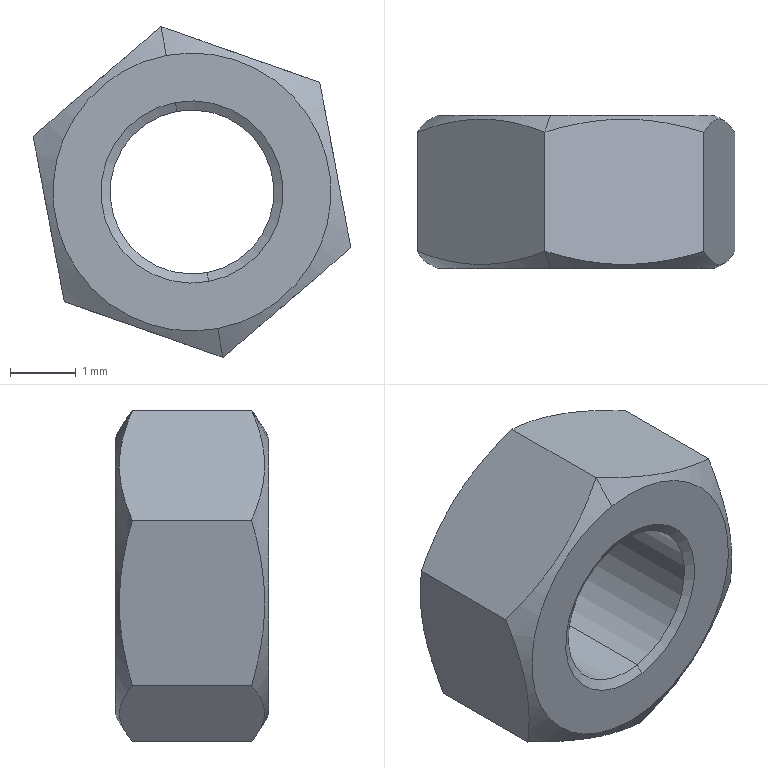Component | SolidWorks | hex nuts, style 1-grades ab gb1-10 | 1 solid | 18 faces | box 4.84 x 2.33 x 5.04 mm | volume 28 mm3 | cone 8 | plane 8 | cylinder 2 | commonest cylinder face diameters 2.5 x2
STEP:
#1=COLOUR_RGB('',0.7922,0.8196,0.9333);
#2=FILL_AREA_STYLE_COLOUR('',#1);
#3=FILL_AREA_STYLE('',(#2));
#4=SURFACE_STYLE_FILL_AREA(#3);
#5=SURFACE_SIDE_STYLE('',(#4));
#6=SURFACE_STYLE_USAGE(.BOTH.,#5);
#7=PRESENTATION_STYLE_ASSIGNMENT((#6));
#8=CARTESIAN_POINT('',(1.085,-0.2477,2.73));
#9=VERTEX_POINT('',#8);
#10=CARTESIAN_POINT('',(1.067,-0.2477,2.827));
#11=VERTEX_POINT('',#10);
#12=CARTESIAN_POINT('',(1.076,-0.2477,2.779));
#13=DIRECTION('',(-0.,-1.,-0.));
#14=DIRECTION('',(-0.1846,0.,0.9828));
#15=AXIS2_PLACEMENT_3D('',#12,#13,#14);
#16=CIRCLE('',#15,0.04921);
#17=EDGE_CURVE('',#9,#11,#16,.T.);
#18=ORIENTED_EDGE('',*,*,#17,.F.);
#19=CARTESIAN_POINT('',(1.086,-0.2509,2.725));
#20=VERTEX_POINT('',#19);
#21=CARTESIAN_POINT('',(1.085,-0.2477,2.73));
#22=DIRECTION('',(0.1598,-0.5,-0.8511));
#23=VECTOR('',#22,39.37);
#24=LINE('',#21,#23);
#25=EDGE_CURVE('',#9,#20,#24,.T.);
#26=ORIENTED_EDGE('',*,*,#25,.T.);
#27=CARTESIAN_POINT('',(1.066,-0.2509,2.833));
#28=VERTEX_POINT('',#27);
#29=CARTESIAN_POINT('',(1.076,-0.2509,2.779));
#30=DIRECTION('',(0.,1.,0.));
#31=DIRECTION('',(-0.1846,0.,0.9828));
#32=AXIS2_PLACEMENT_3D('',#29,#30,#31);
#33=CIRCLE('',#32,0.05468);
#34=EDGE_CURVE('',#28,#20,#33,.T.);
#35=ORIENTED_EDGE('',*,*,#34,.F.);
#36=CARTESIAN_POINT('',(1.067,-0.2477,2.827));
#37=DIRECTION('',(-0.1598,-0.5,0.8511));
#38=VECTOR('',#37,39.37);
#39=LINE('',#36,#38);
#40=EDGE_CURVE('',#11,#28,#39,.T.);
#41=ORIENTED_EDGE('',*,*,#40,.F.);
#42=EDGE_LOOP('',(#18,#26,#35,#41));
#43=FACE_OUTER_BOUND('',#42,.T.);
#44=CARTESIAN_POINT('',(1.076,-0.2477,2.779));
#45=DIRECTION('',(-0.,-1.,-0.));
#46=DIRECTION('',(-0.1846,0.,0.9828));
#47=AXIS2_PLACEMENT_3D('',#44,#45,#46);
#48=CONICAL_SURFACE('',#47,0.04921,1.047);
#49=ADVANCED_FACE('',(#43),#48,.F.);
#50=CARTESIAN_POINT('',(1.067,-0.1645,2.827));
#51=VERTEX_POINT('',#50);
#52=CARTESIAN_POINT('',(1.085,-0.1645,2.73));
#53=VERTEX_POINT('',#52);
#54=CARTESIAN_POINT('',(1.076,-0.1645,2.779));
#55=DIRECTION('',(0.,1.,0.));
#56=DIRECTION('',(-0.1846,0.,0.9828));
#57=AXIS2_PLACEMENT_3D('',#54,#55,#56);
#58=CIRCLE('',#57,0.04921);
#59=EDGE_CURVE('',#51,#53,#58,.T.);
#60=ORIENTED_EDGE('',*,*,#59,.F.);
#61=CARTESIAN_POINT('',(1.066,-0.159,2.83));
#62=VERTEX_POINT('',#61);
#63=CARTESIAN_POINT('',(1.066,-0.159,2.83));
#64=DIRECTION('',(-0.09228,0.866,0.4914));
#65=VECTOR('',#64,39.37);
#66=LINE('',#63,#65);
#67=EDGE_CURVE('',#51,#62,#66,.T.);
#68=ORIENTED_EDGE('',*,*,#67,.T.);
#69=CARTESIAN_POINT('',(1.085,-0.159,2.727));
#70=VERTEX_POINT('',#69);
#71=CARTESIAN_POINT('',(1.076,-0.159,2.779));
#72=DIRECTION('',(-0.,-1.,-0.));
#73=DIRECTION('',(-0.1846,0.,0.9828));
#74=AXIS2_PLACEMENT_3D('',#71,#72,#73);
#75=CIRCLE('',#74,0.05237);
#76=EDGE_CURVE('',#70,#62,#75,.T.);
#77=ORIENTED_EDGE('',*,*,#76,.F.);
#78=CARTESIAN_POINT('',(1.085,-0.159,2.727));
#79=DIRECTION('',(0.09228,0.866,-0.4914));
#80=VECTOR('',#79,39.37);
#81=LINE('',#78,#80);
#82=EDGE_CURVE('',#53,#70,#81,.T.);
#83=ORIENTED_EDGE('',*,*,#82,.F.);
#84=EDGE_LOOP('',(#60,#68,#77,#83));
#85=FACE_OUTER_BOUND('',#84,.T.);
#86=CARTESIAN_POINT('',(1.076,-0.159,2.779));
#87=DIRECTION('',(0.,1.,0.));
#88=DIRECTION('',(0.1846,0.,-0.9828));
#89=AXIS2_PLACEMENT_3D('',#86,#87,#88);
#90=CONICAL_SURFACE('',#89,0.05237,0.5236);
#91=ADVANCED_FACE('',(#85),#90,.F.);
#92=CARTESIAN_POINT('',(1.091,-0.2509,2.697));
#93=VERTEX_POINT('',#92);
#94=CARTESIAN_POINT('',(1.06,-0.2509,2.861));
#95=VERTEX_POINT('',#94);
#96=CARTESIAN_POINT('',(1.076,-0.2509,2.779));
#97=DIRECTION('',(0.,1.,0.));
#98=DIRECTION('',(0.1846,0.,-0.9828));
#99=AXIS2_PLACEMENT_3D('',#96,#97,#98);
#100=CIRCLE('',#99,0.08339);
#101=EDGE_CURVE('',#93,#95,#100,.T.);
#102=ORIENTED_EDGE('',*,*,#101,.T.);
#103=CARTESIAN_POINT('',(1.057,-0.2407,2.878));
#104=VERTEX_POINT('',#103);
#105=CARTESIAN_POINT('',(1.06,-0.2509,2.861));
#106=DIRECTION('',(-0.1598,0.5,0.8511));
#107=VECTOR('',#106,39.37);
#108=LINE('',#105,#107);
#109=EDGE_CURVE('',#95,#104,#108,.T.);
#110=ORIENTED_EDGE('',*,*,#109,.T.);
#111=CARTESIAN_POINT('',(0.9805,-0.2407,2.812));
#112=VERTEX_POINT('',#111);
#113=CARTESIAN_POINT('',(1.057,-0.2407,2.878));
#114=CARTESIAN_POINT('',(1.045,-0.2455,2.867));
#115=CARTESIAN_POINT('',(1.032,-0.2485,2.856));
#116=CARTESIAN_POINT('',(1.012,-0.2485,2.84));
#117=CARTESIAN_POINT('',(1.006,-0.2478,2.834));
#118=CARTESIAN_POINT('',(0.9931,-0.245,2.823));
#119=CARTESIAN_POINT('',(0.9868,-0.2431,2.818));
#120=CARTESIAN_POINT('',(0.9805,-0.2407,2.812));
#121=B_SPLINE_CURVE_WITH_KNOTS('',3,(#113,#114,#115,#116,#117,#118,#119,#120),.UNSPECIFIED.,.F.,.F.,(4,2,2,4),(0.00000007,0.001296,0.001944,0.002592),.UNSPECIFIED.);
#122=EDGE_CURVE('',#104,#112,#121,.T.);
#123=ORIENTED_EDGE('',*,*,#122,.T.);
#124=CARTESIAN_POINT('',(0.9992,-0.2407,2.713));
#125=VERTEX_POINT('',#124);
#126=CARTESIAN_POINT('',(0.9805,-0.2407,2.812));
#127=CARTESIAN_POINT('',(0.982,-0.2431,2.804));
#128=CARTESIAN_POINT('',(0.9836,-0.245,2.796));
#129=CARTESIAN_POINT('',(0.9867,-0.2478,2.78));
#130=CARTESIAN_POINT('',(0.9883,-0.2485,2.771));
#131=CARTESIAN_POINT('',(0.9914,-0.2485,2.754));
#132=CARTESIAN_POINT('',(0.993,-0.2478,2.746));
#133=CARTESIAN_POINT('',(0.9961,-0.2451,2.729));
#134=CARTESIAN_POINT('',(0.9977,-0.2431,2.721));
#135=CARTESIAN_POINT('',(0.9992,-0.2407,2.713));
#136=B_SPLINE_CURVE_WITH_KNOTS('',3,(#126,#127,#128,#129,#130,#131,#132,#133,#134,#135),.UNSPECIFIED.,.F.,.F.,(4,2,2,2,4),(0.0009504,0.001598,0.002245,0.002893,0.00354),.UNSPECIFIED.);
#137=EDGE_CURVE('',#112,#125,#136,.T.);
#138=ORIENTED_EDGE('',*,*,#137,.T.);
#139=CARTESIAN_POINT('',(1.094,-0.2407,2.679));
#140=VERTEX_POINT('',#139);
#141=CARTESIAN_POINT('',(0.9992,-0.2407,2.713));
#142=CARTESIAN_POINT('',(1.015,-0.2455,2.708));
#143=CARTESIAN_POINT('',(1.031,-0.2485,2.702));
#144=CARTESIAN_POINT('',(1.055,-0.2485,2.693));
#145=CARTESIAN_POINT('',(1.063,-0.2478,2.691));
#146=CARTESIAN_POINT('',(1.079,-0.245,2.685));
#147=CARTESIAN_POINT('',(1.087,-0.2431,2.682));
#148=CARTESIAN_POINT('',(1.094,-0.2407,2.679));
#149=B_SPLINE_CURVE_WITH_KNOTS('',3,(#141,#142,#143,#144,#145,#146,#147,#148),.UNSPECIFIED.,.F.,.F.,(4,2,2,4),(0.00000007,0.001296,0.001944,0.002592),.UNSPECIFIED.);
#150=EDGE_CURVE('',#125,#140,#149,.T.);
#151=ORIENTED_EDGE('',*,*,#150,.T.);
#152=CARTESIAN_POINT('',(1.091,-0.2509,2.697));
#153=DIRECTION('',(0.1598,0.5,-0.8511));
#154=VECTOR('',#153,39.37);
#155=LINE('',#152,#154);
#156=EDGE_CURVE('',#93,#140,#155,.T.);
#157=ORIENTED_EDGE('',*,*,#156,.F.);
#158=EDGE_LOOP('',(#102,#110,#123,#138,#151,#157));
#159=FACE_OUTER_BOUND('',#158,.T.);
#160=CARTESIAN_POINT('',(1.076,-0.2509,2.779));
#161=DIRECTION('',(0.,1.,0.));
#162=DIRECTION('',(0.1846,0.,-0.9828));
#163=AXIS2_PLACEMENT_3D('',#160,#161,#162);
#164=CONICAL_SURFACE('',#163,0.08339,1.047);
#165=ADVANCED_FACE('',(#159),#164,.T.);
#166=CARTESIAN_POINT('',(1.091,-0.159,2.697));
#167=VERTEX_POINT('',#166);
#168=CARTESIAN_POINT('',(1.06,-0.159,2.861));
#169=VERTEX_POINT('',#168);
#170=CARTESIAN_POINT('',(1.076,-0.159,2.779));
#171=DIRECTION('',(0.,1.,0.));
#172=DIRECTION('',(0.1846,0.,-0.9828));
#173=AXIS2_PLACEMENT_3D('',#170,#171,#172);
#174=CIRCLE('',#173,0.08339);
#175=EDGE_CURVE('',#167,#169,#174,.T.);
#176=ORIENTED_EDGE('',*,*,#175,.F.);
#177=CARTESIAN_POINT('',(1.094,-0.1692,2.679));
#178=VERTEX_POINT('',#177);
#179=CARTESIAN_POINT('',(1.094,-0.1692,2.679));
#180=DIRECTION('',(0.1598,-0.5,-0.8511));
#181=VECTOR('',#180,39.37);
#182=LINE('',#179,#181);
#183=EDGE_CURVE('',#167,#178,#182,.T.);
#184=ORIENTED_EDGE('',*,*,#183,.T.);
#185=CARTESIAN_POINT('',(0.9992,-0.1692,2.713));
#186=VERTEX_POINT('',#185);
#187=CARTESIAN_POINT('',(1.094,-0.1692,2.679));
#188=CARTESIAN_POINT('',(1.079,-0.1644,2.685));
#189=CARTESIAN_POINT('',(1.063,-0.1614,2.691));
#190=CARTESIAN_POINT('',(1.039,-0.1614,2.699));
#191=CARTESIAN_POINT('',(1.031,-0.1621,2.702));
#192=CARTESIAN_POINT('',(1.015,-0.1648,2.707));
#193=CARTESIAN_POINT('',(1.007,-0.1668,2.71));
#194=CARTESIAN_POINT('',(0.9992,-0.1692,2.713));
#195=B_SPLINE_CURVE_WITH_KNOTS('',3,(#187,#188,#189,#190,#191,#192,#193,#194),.UNSPECIFIED.,.F.,.F.,(4,2,2,4),(0.00000007,0.001296,0.001944,0.002592),.UNSPECIFIED.);
#196=EDGE_CURVE('',#178,#186,#195,.T.);
#197=ORIENTED_EDGE('',*,*,#196,.T.);
#198=CARTESIAN_POINT('',(0.9805,-0.1692,2.812));
#199=VERTEX_POINT('',#198);
#200=CARTESIAN_POINT('',(0.9992,-0.1692,2.713));
#201=CARTESIAN_POINT('',(0.9977,-0.1668,2.721));
#202=CARTESIAN_POINT('',(0.9961,-0.1648,2.729));
#203=CARTESIAN_POINT('',(0.993,-0.1621,2.746));
#204=CARTESIAN_POINT('',(0.9914,-0.1614,2.754));
#205=CARTESIAN_POINT('',(0.9883,-0.1614,2.771));
#206=CARTESIAN_POINT('',(0.9867,-0.1621,2.78));
#207=CARTESIAN_POINT('',(0.9836,-0.1649,2.796));
#208=CARTESIAN_POINT('',(0.982,-0.1668,2.804));
#209=CARTESIAN_POINT('',(0.9805,-0.1692,2.812));
#210=B_SPLINE_CURVE_WITH_KNOTS('',3,(#200,#201,#202,#203,#204,#205,#206,#207,#208,#209),.UNSPECIFIED.,.F.,.F.,(4,2,2,2,4),(0.00228,0.002929,0.003578,0.004227,0.004876),.UNSPECIFIED.);
#211=EDGE_CURVE('',#186,#199,#210,.T.);
#212=ORIENTED_EDGE('',*,*,#211,.T.);
#213=CARTESIAN_POINT('',(1.057,-0.1692,2.878));
#214=VERTEX_POINT('',#213);
#215=CARTESIAN_POINT('',(0.9805,-0.1692,2.812));
#216=CARTESIAN_POINT('',(0.993,-0.1644,2.823));
#217=CARTESIAN_POINT('',(1.006,-0.1614,2.834));
#218=CARTESIAN_POINT('',(1.025,-0.1614,2.851));
#219=CARTESIAN_POINT('',(1.032,-0.1621,2.856));
#220=CARTESIAN_POINT('',(1.045,-0.1648,2.867));
#221=CARTESIAN_POINT('',(1.051,-0.1668,2.873));
#222=CARTESIAN_POINT('',(1.057,-0.1692,2.878));
#223=B_SPLINE_CURVE_WITH_KNOTS('',3,(#215,#216,#217,#218,#219,#220,#221,#222),.UNSPECIFIED.,.F.,.F.,(4,2,2,4),(0.00000007,0.001296,0.001944,0.002592),.UNSPECIFIED.);
#224=EDGE_CURVE('',#199,#214,#223,.T.);
#225=ORIENTED_EDGE('',*,*,#224,.T.);
#226=CARTESIAN_POINT('',(1.057,-0.1692,2.878));
#227=DIRECTION('',(-0.1598,-0.5,0.8511));
#228=VECTOR('',#227,39.37);
#229=LINE('',#226,#228);
#230=EDGE_CURVE('',#169,#214,#229,.T.);
#231=ORIENTED_EDGE('',*,*,#230,.F.);
#232=EDGE_LOOP('',(#176,#184,#197,#212,#225,#231));
#233=FACE_OUTER_BOUND('',#232,.T.);
#234=CARTESIAN_POINT('',(1.076,-0.1692,2.779));
#235=DIRECTION('',(-0.,-1.,-0.));
#236=DIRECTION('',(-0.1846,0.,0.9828));
#237=AXIS2_PLACEMENT_3D('',#234,#235,#236);
#238=CONICAL_SURFACE('',#237,0.101,1.047);
#239=ADVANCED_FACE('',(#233),#238,.T.);
#240=ORIENTED_EDGE('',*,*,#59,.T.);
#241=CARTESIAN_POINT('',(1.085,-0.159,2.73));
#242=DIRECTION('',(-0.,-1.,-0.));
#243=VECTOR('',#242,39.37);
#244=LINE('',#241,#243);
#245=EDGE_CURVE('',#53,#9,#244,.T.);
#246=ORIENTED_EDGE('',*,*,#245,.T.);
#247=ORIENTED_EDGE('',*,*,#17,.T.);
#248=CARTESIAN_POINT('',(1.067,-0.159,2.827));
#249=DIRECTION('',(-0.,-1.,-0.));
#250=VECTOR('',#249,39.37);
#251=LINE('',#248,#250);
#252=EDGE_CURVE('',#51,#11,#251,.T.);
#253=ORIENTED_EDGE('',*,*,#252,.F.);
#254=EDGE_LOOP('',(#240,#246,#247,#253));
#255=FACE_OUTER_BOUND('',#254,.T.);
#256=CARTESIAN_POINT('',(1.076,-0.159,2.779));
#257=DIRECTION('',(-0.,-1.,-0.));
#258=DIRECTION('',(-0.1846,0.,0.9828));
#259=AXIS2_PLACEMENT_3D('',#256,#257,#258);
#260=CYLINDRICAL_SURFACE('',#259,0.04921);
#261=ADVANCED_FACE('',(#255),#260,.F.);
#262=CARTESIAN_POINT('',(1.152,-0.2407,2.845));
#263=VERTEX_POINT('',#262);
#264=CARTESIAN_POINT('',(1.152,-0.2407,2.845));
#265=CARTESIAN_POINT('',(1.137,-0.2455,2.85));
#266=CARTESIAN_POINT('',(1.121,-0.2485,2.856));
#267=CARTESIAN_POINT('',(1.097,-0.2485,2.864));
#268=CARTESIAN_POINT('',(1.089,-0.2478,2.867));
#269=CARTESIAN_POINT('',(1.073,-0.245,2.873));
#270=CARTESIAN_POINT('',(1.065,-0.2431,2.875));
#271=CARTESIAN_POINT('',(1.057,-0.2407,2.878));
#272=B_SPLINE_CURVE_WITH_KNOTS('',3,(#264,#265,#266,#267,#268,#269,#270,#271),.UNSPECIFIED.,.F.,.F.,(4,2,2,4),(0.00000007,0.001296,0.001944,0.002592),.UNSPECIFIED.);
#273=EDGE_CURVE('',#263,#104,#272,.T.);
#274=ORIENTED_EDGE('',*,*,#273,.F.);
#275=CARTESIAN_POINT('',(1.152,-0.1692,2.845));
#276=VERTEX_POINT('',#275);
#277=CARTESIAN_POINT('',(1.152,-0.159,2.845));
#278=DIRECTION('',(-0.,-1.,-0.));
#279=VECTOR('',#278,39.37);
#280=LINE('',#277,#279);
#281=EDGE_CURVE('',#276,#263,#280,.T.);
#282=ORIENTED_EDGE('',*,*,#281,.F.);
#283=CARTESIAN_POINT('',(1.057,-0.1692,2.878));
#284=CARTESIAN_POINT('',(1.073,-0.1644,2.873));
#285=CARTESIAN_POINT('',(1.089,-0.1614,2.867));
#286=CARTESIAN_POINT('',(1.113,-0.1614,2.859));
#287=CARTESIAN_POINT('',(1.121,-0.1621,2.856));
#288=CARTESIAN_POINT('',(1.137,-0.1648,2.85));
#289=CARTESIAN_POINT('',(1.145,-0.1668,2.847));
#290=CARTESIAN_POINT('',(1.152,-0.1692,2.845));
#291=B_SPLINE_CURVE_WITH_KNOTS('',3,(#283,#284,#285,#286,#287,#288,#289,#290),.UNSPECIFIED.,.F.,.F.,(4,2,2,4),(0.00000007,0.001296,0.001944,0.002592),.UNSPECIFIED.);
#292=EDGE_CURVE('',#214,#276,#291,.T.);
#293=ORIENTED_EDGE('',*,*,#292,.F.);
#294=CARTESIAN_POINT('',(1.057,-0.159,2.878));
#295=DIRECTION('',(-0.,-1.,-0.));
#296=VECTOR('',#295,39.37);
#297=LINE('',#294,#296);
#298=EDGE_CURVE('',#214,#104,#297,.T.);
#299=ORIENTED_EDGE('',*,*,#298,.T.);
#300=EDGE_LOOP('',(#274,#282,#293,#299));
#301=FACE_OUTER_BOUND('',#300,.T.);
#302=CARTESIAN_POINT('',(1.152,-0.159,2.845));
#303=DIRECTION('',(0.3316,0.,0.9434));
#304=DIRECTION('',(-0.9434,0.,0.3316));
#305=AXIS2_PLACEMENT_3D('',#302,#303,#304);
#306=PLANE('',#305);
#307=ADVANCED_FACE('',(#301),#306,.T.);
#308=CARTESIAN_POINT('',(1.171,-0.2407,2.745));
#309=VERTEX_POINT('',#308);
#310=CARTESIAN_POINT('',(1.171,-0.2407,2.745));
#311=CARTESIAN_POINT('',(1.17,-0.2431,2.753));
#312=CARTESIAN_POINT('',(1.168,-0.2451,2.762));
#313=CARTESIAN_POINT('',(1.165,-0.2478,2.778));
#314=CARTESIAN_POINT('',(1.163,-0.2485,2.787));
#315=CARTESIAN_POINT('',(1.16,-0.2485,2.803));
#316=CARTESIAN_POINT('',(1.159,-0.2478,2.812));
#317=CARTESIAN_POINT('',(1.156,-0.245,2.828));
#318=CARTESIAN_POINT('',(1.154,-0.2431,2.837));
#319=CARTESIAN_POINT('',(1.152,-0.2407,2.845));
#320=B_SPLINE_CURVE_WITH_KNOTS('',3,(#310,#311,#312,#313,#314,#315,#316,#317,#318,#319),.UNSPECIFIED.,.F.,.F.,(4,2,2,2,4),(0.00228,0.002929,0.003578,0.004227,0.004876),.UNSPECIFIED.);
#321=EDGE_CURVE('',#309,#263,#320,.T.);
#322=ORIENTED_EDGE('',*,*,#321,.F.);
#323=CARTESIAN_POINT('',(1.171,-0.1692,2.745));
#324=VERTEX_POINT('',#323);
#325=CARTESIAN_POINT('',(1.171,-0.159,2.745));
#326=DIRECTION('',(-0.,-1.,-0.));
#327=VECTOR('',#326,39.37);
#328=LINE('',#325,#327);
#329=EDGE_CURVE('',#324,#309,#328,.T.);
#330=ORIENTED_EDGE('',*,*,#329,.F.);
#331=CARTESIAN_POINT('',(1.152,-0.1692,2.845));
#332=CARTESIAN_POINT('',(1.154,-0.1668,2.837));
#333=CARTESIAN_POINT('',(1.156,-0.1649,2.828));
#334=CARTESIAN_POINT('',(1.159,-0.1621,2.812));
#335=CARTESIAN_POINT('',(1.16,-0.1614,2.803));
#336=CARTESIAN_POINT('',(1.163,-0.1614,2.787));
#337=CARTESIAN_POINT('',(1.165,-0.1621,2.778));
#338=CARTESIAN_POINT('',(1.168,-0.1648,2.762));
#339=CARTESIAN_POINT('',(1.17,-0.1668,2.753));
#340=CARTESIAN_POINT('',(1.171,-0.1692,2.745));
#341=B_SPLINE_CURVE_WITH_KNOTS('',3,(#331,#332,#333,#334,#335,#336,#337,#338,#339,#340),.UNSPECIFIED.,.F.,.F.,(4,2,2,2,4),(0.0009504,0.001598,0.002245,0.002893,0.00354),.UNSPECIFIED.);
#342=EDGE_CURVE('',#276,#324,#341,.T.);
#343=ORIENTED_EDGE('',*,*,#342,.F.);
#344=ORIENTED_EDGE('',*,*,#281,.T.);
#345=EDGE_LOOP('',(#322,#330,#343,#344));
#346=FACE_OUTER_BOUND('',#345,.T.);
#347=CARTESIAN_POINT('',(1.171,-0.159,2.745));
#348=DIRECTION('',(0.9828,-0.,0.1846));
#349=DIRECTION('',(0.,1.,0.));
#350=AXIS2_PLACEMENT_3D('',#347,#348,#349);
#351=PLANE('',#350);
#352=ADVANCED_FACE('',(#346),#351,.T.);
#353=CARTESIAN_POINT('',(1.094,-0.2407,2.679));
#354=CARTESIAN_POINT('',(1.107,-0.2455,2.69));
#355=CARTESIAN_POINT('',(1.12,-0.2485,2.701));
#356=CARTESIAN_POINT('',(1.139,-0.2485,2.718));
#357=CARTESIAN_POINT('',(1.146,-0.2478,2.724));
#358=CARTESIAN_POINT('',(1.159,-0.245,2.734));
#359=CARTESIAN_POINT('',(1.165,-0.2431,2.74));
#360=CARTESIAN_POINT('',(1.171,-0.2407,2.745));
#361=B_SPLINE_CURVE_WITH_KNOTS('',3,(#353,#354,#355,#356,#357,#358,#359,#360),.UNSPECIFIED.,.F.,.F.,(4,2,2,4),(0.00000007,0.001296,0.001944,0.002592),.UNSPECIFIED.);
#362=EDGE_CURVE('',#140,#309,#361,.T.);
#363=ORIENTED_EDGE('',*,*,#362,.F.);
#364=CARTESIAN_POINT('',(1.094,-0.159,2.679));
#365=DIRECTION('',(-0.,-1.,-0.));
#366=VECTOR('',#365,39.37);
#367=LINE('',#364,#366);
#368=EDGE_CURVE('',#178,#140,#367,.T.);
#369=ORIENTED_EDGE('',*,*,#368,.F.);
#370=CARTESIAN_POINT('',(1.171,-0.1692,2.745));
#371=CARTESIAN_POINT('',(1.159,-0.1644,2.735));
#372=CARTESIAN_POINT('',(1.146,-0.1614,2.724));
#373=CARTESIAN_POINT('',(1.126,-0.1614,2.707));
#374=CARTESIAN_POINT('',(1.12,-0.1621,2.701));
#375=CARTESIAN_POINT('',(1.107,-0.1648,2.69));
#376=CARTESIAN_POINT('',(1.101,-0.1668,2.685));
#377=CARTESIAN_POINT('',(1.094,-0.1692,2.679));
#378=B_SPLINE_CURVE_WITH_KNOTS('',3,(#370,#371,#372,#373,#374,#375,#376,#377),.UNSPECIFIED.,.F.,.F.,(4,2,2,4),(0.00000007,0.001296,0.001944,0.002592),.UNSPECIFIED.);
#379=EDGE_CURVE('',#324,#178,#378,.T.);
#380=ORIENTED_EDGE('',*,*,#379,.F.);
#381=ORIENTED_EDGE('',*,*,#329,.T.);
#382=EDGE_LOOP('',(#363,#369,#380,#381));
#383=FACE_OUTER_BOUND('',#382,.T.);
#384=CARTESIAN_POINT('',(1.094,-0.159,2.679));
#385=DIRECTION('',(0.6512,-0.,-0.7589));
#386=DIRECTION('',(0.7589,-0.,0.6512));
#387=AXIS2_PLACEMENT_3D('',#384,#385,#386);
#388=PLANE('',#387);
#389=ADVANCED_FACE('',(#383),#388,.T.);
#390=ORIENTED_EDGE('',*,*,#150,.F.);
#391=CARTESIAN_POINT('',(0.9992,-0.159,2.713));
#392=DIRECTION('',(-0.,-1.,-0.));
#393=VECTOR('',#392,39.37);
#394=LINE('',#391,#393);
#395=EDGE_CURVE('',#186,#125,#394,.T.);
#396=ORIENTED_EDGE('',*,*,#395,.F.);
#397=ORIENTED_EDGE('',*,*,#196,.F.);
#398=ORIENTED_EDGE('',*,*,#368,.T.);
#399=EDGE_LOOP('',(#390,#396,#397,#398));
#400=FACE_OUTER_BOUND('',#399,.T.);
#401=CARTESIAN_POINT('',(0.9992,-0.159,2.713));
#402=DIRECTION('',(-0.3316,-0.,-0.9434));
#403=DIRECTION('',(0.9434,-0.,-0.3316));
#404=AXIS2_PLACEMENT_3D('',#401,#402,#403);
#405=PLANE('',#404);
#406=ADVANCED_FACE('',(#400),#405,.T.);
#407=ORIENTED_EDGE('',*,*,#137,.F.);
#408=CARTESIAN_POINT('',(0.9805,-0.159,2.812));
#409=DIRECTION('',(-0.,-1.,-0.));
#410=VECTOR('',#409,39.37);
#411=LINE('',#408,#410);
#412=EDGE_CURVE('',#199,#112,#411,.T.);
#413=ORIENTED_EDGE('',*,*,#412,.F.);
#414=ORIENTED_EDGE('',*,*,#211,.F.);
#415=ORIENTED_EDGE('',*,*,#395,.T.);
#416=EDGE_LOOP('',(#407,#413,#414,#415));
#417=FACE_OUTER_BOUND('',#416,.T.);
#418=CARTESIAN_POINT('',(0.9805,-0.159,2.812));
#419=DIRECTION('',(-0.9828,0.,-0.1846));
#420=DIRECTION('',(-0.,-1.,-0.));
#421=AXIS2_PLACEMENT_3D('',#418,#419,#420);
#422=PLANE('',#421);
#423=ADVANCED_FACE('',(#417),#422,.T.);
#424=ORIENTED_EDGE('',*,*,#122,.F.);
#425=ORIENTED_EDGE('',*,*,#298,.F.);
#426=ORIENTED_EDGE('',*,*,#224,.F.);
#427=ORIENTED_EDGE('',*,*,#412,.T.);
#428=EDGE_LOOP('',(#424,#425,#426,#427));
#429=FACE_OUTER_BOUND('',#428,.T.);
#430=CARTESIAN_POINT('',(1.057,-0.159,2.878));
#431=DIRECTION('',(-0.6512,0.,0.7589));
#432=DIRECTION('',(-0.7589,0.,-0.6512));
#433=AXIS2_PLACEMENT_3D('',#430,#431,#432);
#434=PLANE('',#433);
#435=ADVANCED_FACE('',(#429),#434,.T.);
#436=ORIENTED_EDGE('',*,*,#76,.T.);
#437=CARTESIAN_POINT('',(1.076,-0.159,2.779));
#438=DIRECTION('',(-0.,-1.,-0.));
#439=DIRECTION('',(-0.1846,0.,0.9828));
#440=AXIS2_PLACEMENT_3D('',#437,#438,#439);
#441=CIRCLE('',#440,0.05237);
#442=EDGE_CURVE('',#62,#70,#441,.T.);
#443=ORIENTED_EDGE('',*,*,#442,.T.);
#444=EDGE_LOOP('',(#436,#443));
#445=FACE_BOUND('',#444,.T.);
#446=CARTESIAN_POINT('',(1.076,-0.159,2.779));
#447=DIRECTION('',(0.,1.,0.));
#448=DIRECTION('',(0.1846,0.,-0.9828));
#449=AXIS2_PLACEMENT_3D('',#446,#447,#448);
#450=CIRCLE('',#449,0.08339);
#451=EDGE_CURVE('',#169,#167,#450,.T.);
#452=ORIENTED_EDGE('',*,*,#451,.T.);
#453=ORIENTED_EDGE('',*,*,#175,.T.);
#454=EDGE_LOOP('',(#452,#453));
#455=FACE_OUTER_BOUND('',#454,.T.);
#456=CARTESIAN_POINT('',(1.057,-0.159,2.878));
#457=DIRECTION('',(-0.,-1.,0.));
#458=DIRECTION('',(-0.1846,0.,0.9828));
#459=AXIS2_PLACEMENT_3D('',#456,#457,#458);
#460=PLANE('',#459);
#461=ADVANCED_FACE('',(#445,#455),#460,.F.);
#462=ORIENTED_EDGE('',*,*,#34,.T.);
#463=CARTESIAN_POINT('',(1.076,-0.2509,2.779));
#464=DIRECTION('',(0.,1.,0.));
#465=DIRECTION('',(-0.1846,0.,0.9828));
#466=AXIS2_PLACEMENT_3D('',#463,#464,#465);
#467=CIRCLE('',#466,0.05468);
#468=EDGE_CURVE('',#20,#28,#467,.T.);
#469=ORIENTED_EDGE('',*,*,#468,.T.);
#470=EDGE_LOOP('',(#462,#469));
#471=FACE_BOUND('',#470,.T.);
#472=ORIENTED_EDGE('',*,*,#101,.F.);
#473=CARTESIAN_POINT('',(1.076,-0.2509,2.779));
#474=DIRECTION('',(0.,1.,0.));
#475=DIRECTION('',(0.1846,0.,-0.9828));
#476=AXIS2_PLACEMENT_3D('',#473,#474,#475);
#477=CIRCLE('',#476,0.08339);
#478=EDGE_CURVE('',#95,#93,#477,.T.);
#479=ORIENTED_EDGE('',*,*,#478,.F.);
#480=EDGE_LOOP('',(#472,#479));
#481=FACE_OUTER_BOUND('',#480,.T.);
#482=CARTESIAN_POINT('',(1.057,-0.2509,2.878));
#483=DIRECTION('',(-0.,-1.,0.));
#484=DIRECTION('',(-0.1846,0.,0.9828));
#485=AXIS2_PLACEMENT_3D('',#482,#483,#484);
#486=PLANE('',#485);
#487=ADVANCED_FACE('',(#471,#481),#486,.T.);
#488=ORIENTED_EDGE('',*,*,#245,.F.);
#489=CARTESIAN_POINT('',(1.076,-0.1645,2.779));
#490=DIRECTION('',(0.,1.,0.));
#491=DIRECTION('',(-0.1846,0.,0.9828));
#492=AXIS2_PLACEMENT_3D('',#489,#490,#491);
#493=CIRCLE('',#492,0.04921);
#494=EDGE_CURVE('',#53,#51,#493,.T.);
#495=ORIENTED_EDGE('',*,*,#494,.T.);
#496=ORIENTED_EDGE('',*,*,#252,.T.);
#497=CARTESIAN_POINT('',(1.076,-0.2477,2.779));
#498=DIRECTION('',(-0.,-1.,-0.));
#499=DIRECTION('',(-0.1846,0.,0.9828));
#500=AXIS2_PLACEMENT_3D('',#497,#498,#499);
#501=CIRCLE('',#500,0.04921);
#502=EDGE_CURVE('',#11,#9,#501,.T.);
#503=ORIENTED_EDGE('',*,*,#502,.T.);
#504=EDGE_LOOP('',(#488,#495,#496,#503));
#505=FACE_OUTER_BOUND('',#504,.T.);
#506=CARTESIAN_POINT('',(1.076,-0.159,2.779));
#507=DIRECTION('',(-0.,-1.,-0.));
#508=DIRECTION('',(-0.1846,0.,0.9828));
#509=AXIS2_PLACEMENT_3D('',#506,#507,#508);
#510=CYLINDRICAL_SURFACE('',#509,0.04921);
#511=ADVANCED_FACE('',(#505),#510,.F.);
#512=ORIENTED_EDGE('',*,*,#183,.F.);
#513=ORIENTED_EDGE('',*,*,#451,.F.);
#514=ORIENTED_EDGE('',*,*,#230,.T.);
#515=ORIENTED_EDGE('',*,*,#292,.T.);
#516=ORIENTED_EDGE('',*,*,#342,.T.);
#517=ORIENTED_EDGE('',*,*,#379,.T.);
#518=EDGE_LOOP('',(#512,#513,#514,#515,#516,#517));
#519=FACE_OUTER_BOUND('',#518,.T.);
#520=CARTESIAN_POINT('',(1.076,-0.1692,2.779));
#521=DIRECTION('',(-0.,-1.,-0.));
#522=DIRECTION('',(-0.1846,0.,0.9828));
#523=AXIS2_PLACEMENT_3D('',#520,#521,#522);
#524=CONICAL_SURFACE('',#523,0.101,1.047);
#525=ADVANCED_FACE('',(#519),#524,.T.);
#526=ORIENTED_EDGE('',*,*,#109,.F.);
#527=ORIENTED_EDGE('',*,*,#478,.T.);
#528=ORIENTED_EDGE('',*,*,#156,.T.);
#529=ORIENTED_EDGE('',*,*,#362,.T.);
#530=ORIENTED_EDGE('',*,*,#321,.T.);
#531=ORIENTED_EDGE('',*,*,#273,.T.);
#532=EDGE_LOOP('',(#526,#527,#528,#529,#530,#531));
#533=FACE_OUTER_BOUND('',#532,.T.);
#534=CARTESIAN_POINT('',(1.076,-0.2509,2.779));
#535=DIRECTION('',(0.,1.,0.));
#536=DIRECTION('',(0.1846,0.,-0.9828));
#537=AXIS2_PLACEMENT_3D('',#534,#535,#536);
#538=CONICAL_SURFACE('',#537,0.08339,1.047);
#539=ADVANCED_FACE('',(#533),#538,.T.);
#540=ORIENTED_EDGE('',*,*,#67,.F.);
#541=ORIENTED_EDGE('',*,*,#494,.F.);
#542=ORIENTED_EDGE('',*,*,#82,.T.);
#543=ORIENTED_EDGE('',*,*,#442,.F.);
#544=EDGE_LOOP('',(#540,#541,#542,#543));
#545=FACE_OUTER_BOUND('',#544,.T.);
#546=CARTESIAN_POINT('',(1.076,-0.159,2.779));
#547=DIRECTION('',(0.,1.,0.));
#548=DIRECTION('',(0.1846,0.,-0.9828));
#549=AXIS2_PLACEMENT_3D('',#546,#547,#548);
#550=CONICAL_SURFACE('',#549,0.05237,0.5236);
#551=ADVANCED_FACE('',(#545),#550,.F.);
#552=ORIENTED_EDGE('',*,*,#25,.F.);
#553=ORIENTED_EDGE('',*,*,#502,.F.);
#554=ORIENTED_EDGE('',*,*,#40,.T.);
#555=ORIENTED_EDGE('',*,*,#468,.F.);
#556=EDGE_LOOP('',(#552,#553,#554,#555));
#557=FACE_OUTER_BOUND('',#556,.T.);
#558=CARTESIAN_POINT('',(1.076,-0.2477,2.779));
#559=DIRECTION('',(-0.,-1.,-0.));
#560=DIRECTION('',(-0.1846,0.,0.9828));
#561=AXIS2_PLACEMENT_3D('',#558,#559,#560);
#562=CONICAL_SURFACE('',#561,0.04921,1.047);
#563=ADVANCED_FACE('',(#557),#562,.F.);
#564=CLOSED_SHELL('',(#49,#91,#165,#239,#261,#307,#352,#389,#406,#423,#435,#461,#487,#511,#525,#539,#551,#563));
#565=MANIFOLD_SOLID_BREP('',#564);
#566=STYLED_ITEM('',(#7),#565);
#567=PRESENTATION_LAYER_ASSIGNMENT('','',(#566));
#568=(LENGTH_UNIT()NAMED_UNIT(*)SI_UNIT($,.METRE.));
#569=LENGTH_MEASURE_WITH_UNIT(LENGTH_MEASURE(0.0254),#568);
#570=DIMENSIONAL_EXPONENTS(1.,0.,0.,0.,0.,0.,0.);
#571=(CONVERSION_BASED_UNIT('',#569)LENGTH_UNIT()NAMED_UNIT(#570));
#572=UNCERTAINTY_MEASURE_WITH_UNIT(LENGTH_MEASURE(0.00001),#571,'','');
#573=(NAMED_UNIT(*)PLANE_ANGLE_UNIT()SI_UNIT($,.RADIAN.));
#574=(NAMED_UNIT(*)SI_UNIT($,.STERADIAN.)SOLID_ANGLE_UNIT());
#575=(GEOMETRIC_REPRESENTATION_CONTEXT(3)GLOBAL_UNCERTAINTY_ASSIGNED_CONTEXT((#572))GLOBAL_UNIT_ASSIGNED_CONTEXT((#571,#573,#574))REPRESENTATION_CONTEXT('',''));
#576=MECHANICAL_DESIGN_GEOMETRIC_PRESENTATION_REPRESENTATION('',(#566),#575);
#577=CARTESIAN_POINT('',(0.,0.,0.));
#578=DIRECTION('',(0.,0.,1.));
#579=DIRECTION('',(1.,0.,0.));
#580=AXIS2_PLACEMENT_3D('',#577,#578,#579);
#581=(LENGTH_UNIT()NAMED_UNIT(*)SI_UNIT($,.METRE.));
#582=LENGTH_MEASURE_WITH_UNIT(LENGTH_MEASURE(0.0254),#581);
#583=DIMENSIONAL_EXPONENTS(1.,0.,0.,0.,0.,0.,0.);
#584=(CONVERSION_BASED_UNIT('',#582)LENGTH_UNIT()NAMED_UNIT(#583));
#585=UNCERTAINTY_MEASURE_WITH_UNIT(LENGTH_MEASURE(0.00001),#584,'','');
#586=(NAMED_UNIT(*)PLANE_ANGLE_UNIT()SI_UNIT($,.RADIAN.));
#587=(NAMED_UNIT(*)SI_UNIT($,.STERADIAN.)SOLID_ANGLE_UNIT());
#588=(GEOMETRIC_REPRESENTATION_CONTEXT(3)GLOBAL_UNCERTAINTY_ASSIGNED_CONTEXT((#585))GLOBAL_UNIT_ASSIGNED_CONTEXT((#584,#586,#587))REPRESENTATION_CONTEXT('',''));
#589=ADVANCED_BREP_SHAPE_REPRESENTATION('',(#565,#580),#588);